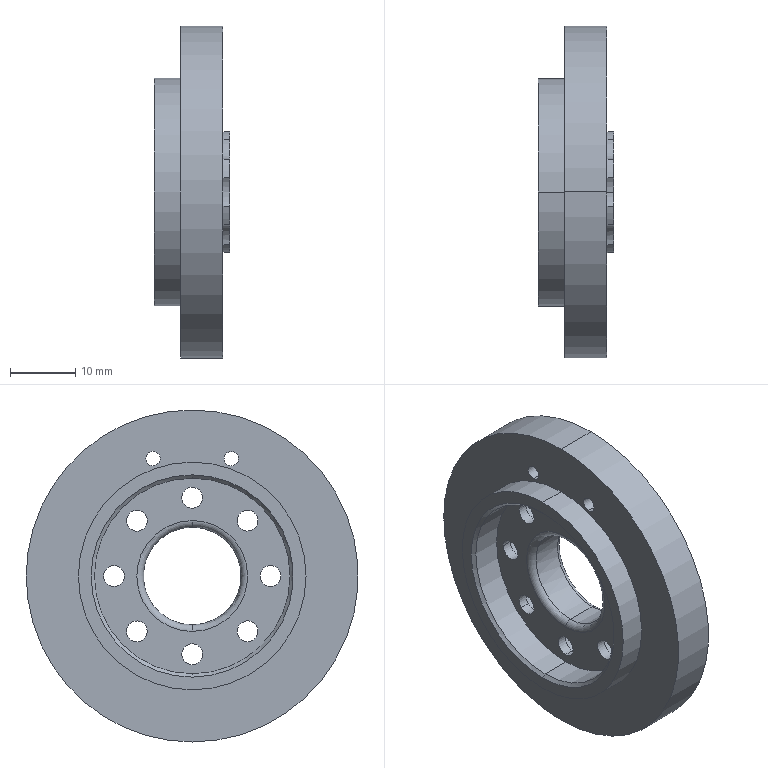CAM job | Mastercam | mm | 4 operations | part box 11.5 x 50.9 x 50.9
1. Contour (Ramp) | 4 - 4 平铣刀
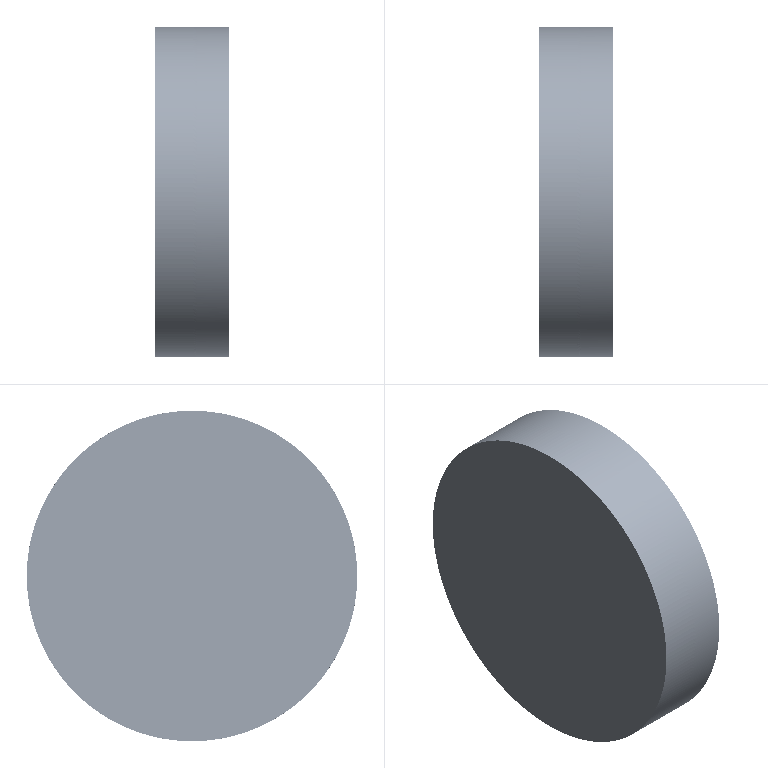2. Contour (2D) | 4 - 4 平铣刀
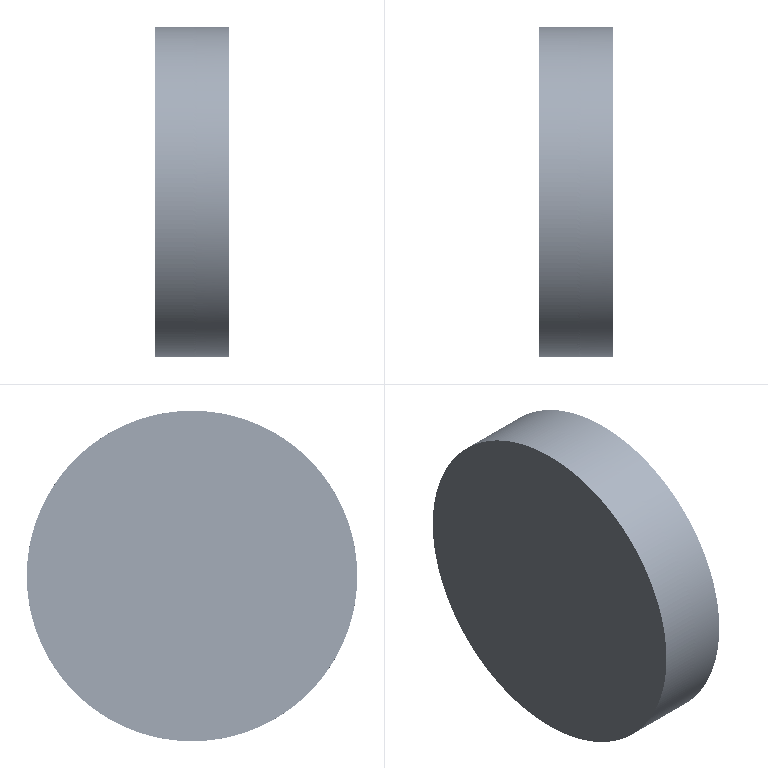3. Drill/Counterbore | 7 - 4 倒角刀
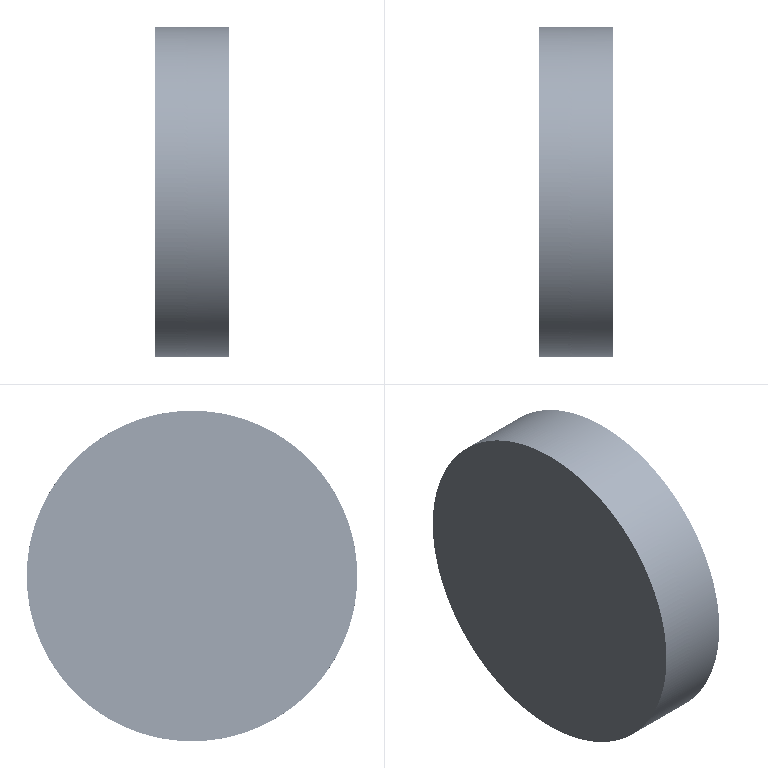4. Deburr 5-axis | 7 - 4 倒角刀